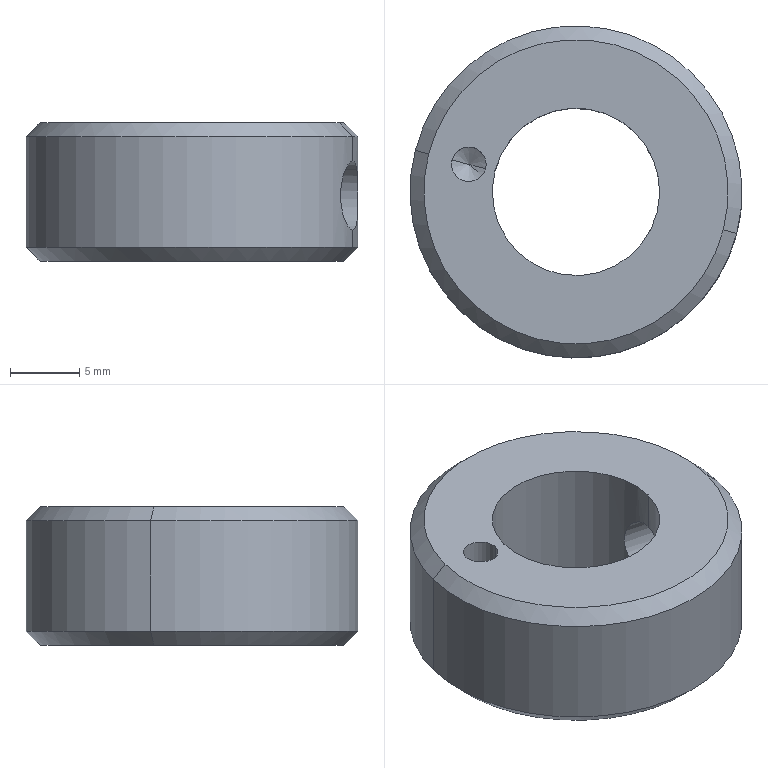Component | SolidWorks | TAR-02-036SpringFixingSleeve-1 | 1 solid | 16 faces | box 24 x 24 x 10 mm | volume 3147 mm3 | cylinder 8 | cone 6 | plane 2 | commonest cylinder face diameters 2.5 x2 5 x2 12.1 x2 24 x2
build123d program:
from build123d import *

# Parameters (mm, degrees)
SKETCH1_R                     = 12
SKETCH1_R_2                   = 6.05
BOSS_EXTRUDE1_DEPTH           = 10
CHAMFER1_SIZE                 = 1
M6_TAPPED_HOLE1_D             = 5
M6_TAPPED_HOLE1_DEPTH         = 12
M6_TAPPED_HOLE1_TIP           = 1.502
SIZE_MM_DOWEL_PIN_HOLE1_D     = 2.5
SIZE_MM_DOWEL_PIN_HOLE1_DEPTH = 7
SIZE_MM_DOWEL_PIN_HOLE1_TIP   = 0.7511


with BuildPart() as part:
    # Sketch1 → Boss-Extrude1 (new body)
    with BuildSketch(Plane.XY):
        Circle(SKETCH1_R)
        Circle(SKETCH1_R_2, mode=Mode.SUBTRACT)
    extrude(amount=BOSS_EXTRUDE1_DEPTH)

    # Chamfer1
    chamfer1_edges = [part.edges().sort_by_distance(p)[0] for p in [
        (-12, 0, 0),
        (-12, 0, 10),
    ]]
    chamfer(chamfer1_edges, length=CHAMFER1_SIZE)

    # M6 Tapped Hole1
    with Locations(Plane(origin=(12, 0, 4.747), x_dir=(0, 1, 0), z_dir=(1, 0, 0))):
        with Locations((0, 0)):
            Hole(M6_TAPPED_HOLE1_D / 2, depth=M6_TAPPED_HOLE1_DEPTH)
            with Locations((0, 0, -(M6_TAPPED_HOLE1_DEPTH + M6_TAPPED_HOLE1_TIP / 2))):  # 118° drill point
                Cone(0, M6_TAPPED_HOLE1_D / 2, M6_TAPPED_HOLE1_TIP, mode=Mode.SUBTRACT)

    # Size mm Dowel Pin Hole1
    with Locations(Plane(origin=(-8, 0, 10), x_dir=(1, 0, 0), z_dir=(0, 0, 1))):
        with Locations((0, 0)):
            Hole(SIZE_MM_DOWEL_PIN_HOLE1_D / 2, depth=SIZE_MM_DOWEL_PIN_HOLE1_DEPTH)
            with Locations((0, 0, -(SIZE_MM_DOWEL_PIN_HOLE1_DEPTH + SIZE_MM_DOWEL_PIN_HOLE1_TIP / 2))):  # 118° drill point
                Cone(0, SIZE_MM_DOWEL_PIN_HOLE1_D / 2, SIZE_MM_DOWEL_PIN_HOLE1_TIP, mode=Mode.SUBTRACT)


solid = part.part

# Placed as in the assembly
solid = solid.moved(Location((-45.891, 68.788, -66.881), (0, 0, -14.47)))
STEP:
#1=COLOUR_RGB('',0.7922,0.8196,0.9333);
#2=FILL_AREA_STYLE_COLOUR('',#1);
#3=FILL_AREA_STYLE('',(#2));
#4=SURFACE_STYLE_FILL_AREA(#3);
#5=SURFACE_SIDE_STYLE('',(#4));
#6=SURFACE_STYLE_USAGE(.BOTH.,#5);
#7=PRESENTATION_STYLE_ASSIGNMENT((#6));
#8=CARTESIAN_POINT('',(-2.159,2.799,-2.515));
#9=VERTEX_POINT('',#8);
#10=CARTESIAN_POINT('',(-2.064,2.775,-2.515));
#11=VERTEX_POINT('',#10);
#12=CARTESIAN_POINT('',(-2.112,2.787,-2.515));
#13=DIRECTION('',(0.,0.,1.));
#14=DIRECTION('',(0.9683,-0.2499,0.));
#15=AXIS2_PLACEMENT_3D('',#12,#13,#14);
#16=CIRCLE('',#15,0.04921);
#17=EDGE_CURVE('',#9,#11,#16,.T.);
#18=ORIENTED_EDGE('',*,*,#17,.F.);
#19=CARTESIAN_POINT('',(-2.159,2.799,-2.239));
#20=VERTEX_POINT('',#19);
#21=CARTESIAN_POINT('',(-2.159,2.799,-2.239));
#22=DIRECTION('',(0.,0.,1.));
#23=VECTOR('',#22,39.37);
#24=LINE('',#21,#23);
#25=EDGE_CURVE('',#9,#20,#24,.T.);
#26=ORIENTED_EDGE('',*,*,#25,.T.);
#27=CARTESIAN_POINT('',(-2.064,2.775,-2.239));
#28=VERTEX_POINT('',#27);
#29=CARTESIAN_POINT('',(-2.112,2.787,-2.239));
#30=DIRECTION('',(0.,0.,1.));
#31=DIRECTION('',(0.9683,-0.2499,0.));
#32=AXIS2_PLACEMENT_3D('',#29,#30,#31);
#33=CIRCLE('',#32,0.04921);
#34=EDGE_CURVE('',#20,#28,#33,.T.);
#35=ORIENTED_EDGE('',*,*,#34,.T.);
#36=CARTESIAN_POINT('',(-2.064,2.775,-2.239));
#37=DIRECTION('',(0.,0.,1.));
#38=VECTOR('',#37,39.37);
#39=LINE('',#36,#38);
#40=EDGE_CURVE('',#11,#28,#39,.T.);
#41=ORIENTED_EDGE('',*,*,#40,.F.);
#42=EDGE_LOOP('',(#18,#26,#35,#41));
#43=FACE_OUTER_BOUND('',#42,.T.);
#44=CARTESIAN_POINT('',(-2.112,2.787,-2.239));
#45=DIRECTION('',(0.,0.,1.));
#46=DIRECTION('',(0.9683,-0.2499,0.));
#47=AXIS2_PLACEMENT_3D('',#44,#45,#46);
#48=CYLINDRICAL_SURFACE('',#47,0.04921);
#49=ADVANCED_FACE('',(#43),#48,.F.);
#50=CARTESIAN_POINT('',(-2.112,2.787,-2.545));
#51=VERTEX_POINT('',#50);
#52=CARTESIAN_POINT('',(-2.064,2.775,-2.515));
#53=DIRECTION('',(0.83,-0.2142,0.515));
#54=VECTOR('',#53,39.37);
#55=LINE('',#52,#54);
#56=EDGE_CURVE('',#51,#11,#55,.T.);
#57=ORIENTED_EDGE('',*,*,#56,.F.);
#58=CARTESIAN_POINT('',(-2.159,2.799,-2.515));
#59=DIRECTION('',(-0.83,0.2142,0.515));
#60=VECTOR('',#59,39.37);
#61=LINE('',#58,#60);
#62=EDGE_CURVE('',#51,#9,#61,.T.);
#63=ORIENTED_EDGE('',*,*,#62,.T.);
#64=ORIENTED_EDGE('',*,*,#17,.T.);
#65=EDGE_LOOP('',(#57,#63,#64));
#66=FACE_OUTER_BOUND('',#65,.T.);
#67=CARTESIAN_POINT('',(-2.112,2.787,-2.515));
#68=DIRECTION('',(0.,0.,1.));
#69=DIRECTION('',(0.9683,-0.2499,0.));
#70=AXIS2_PLACEMENT_3D('',#67,#68,#69);
#71=CONICAL_SURFACE('',#70,0.04921,1.03);
#72=ADVANCED_FACE('',(#66),#71,.F.);
#73=CARTESIAN_POINT('',(-1.576,2.649,-2.545));
#74=VERTEX_POINT('',#73);
#75=CARTESIAN_POINT('',(-1.576,2.649,-2.348));
#76=VERTEX_POINT('',#75);
#77=CARTESIAN_POINT('',(-1.576,2.649,-2.545));
#78=CARTESIAN_POINT('',(-1.578,2.642,-2.545));
#79=CARTESIAN_POINT('',(-1.58,2.636,-2.544));
#80=CARTESIAN_POINT('',(-1.584,2.624,-2.541));
#81=CARTESIAN_POINT('',(-1.586,2.618,-2.54));
#82=CARTESIAN_POINT('',(-1.591,2.607,-2.535));
#83=CARTESIAN_POINT('',(-1.593,2.602,-2.532));
#84=CARTESIAN_POINT('',(-1.599,2.592,-2.524));
#85=CARTESIAN_POINT('',(-1.601,2.588,-2.52));
#86=CARTESIAN_POINT('',(-1.608,2.576,-2.507));
#87=CARTESIAN_POINT('',(-1.613,2.569,-2.496));
#88=CARTESIAN_POINT('',(-1.618,2.563,-2.478));
#89=CARTESIAN_POINT('',(-1.619,2.561,-2.472));
#90=CARTESIAN_POINT('',(-1.621,2.559,-2.459));
#91=CARTESIAN_POINT('',(-1.621,2.559,-2.453));
#92=CARTESIAN_POINT('',(-1.621,2.559,-2.44));
#93=CARTESIAN_POINT('',(-1.621,2.559,-2.433));
#94=CARTESIAN_POINT('',(-1.619,2.561,-2.42));
#95=CARTESIAN_POINT('',(-1.618,2.563,-2.414));
#96=CARTESIAN_POINT('',(-1.615,2.567,-2.402));
#97=CARTESIAN_POINT('',(-1.613,2.57,-2.397));
#98=CARTESIAN_POINT('',(-1.608,2.576,-2.386));
#99=CARTESIAN_POINT('',(-1.606,2.58,-2.381));
#100=CARTESIAN_POINT('',(-1.601,2.588,-2.372));
#101=CARTESIAN_POINT('',(-1.599,2.592,-2.368));
#102=CARTESIAN_POINT('',(-1.593,2.602,-2.361));
#103=CARTESIAN_POINT('',(-1.591,2.607,-2.358));
#104=CARTESIAN_POINT('',(-1.586,2.618,-2.353));
#105=CARTESIAN_POINT('',(-1.584,2.624,-2.351));
#106=CARTESIAN_POINT('',(-1.58,2.636,-2.348));
#107=CARTESIAN_POINT('',(-1.578,2.642,-2.348));
#108=CARTESIAN_POINT('',(-1.576,2.649,-2.348));
#109=B_SPLINE_CURVE_WITH_KNOTS('',3,(#77,#78,#79,#80,#81,#82,#83,#84,#85,#86,#87,#88,#89,#90,#91,#92,#93,#94,#95,#96,#97,#98,#99,#100,#101,#102,#103,#104,#105,#106,#107,#108),.UNSPECIFIED.,.F.,.F.,(4,2,2,2,2,2,2,2,2,2,2,2,2,2,2,4),(0.,0.0004941,0.0009882,0.001482,0.001976,0.002965,0.003459,0.003953,0.004447,0.004941,0.005435,0.005929,0.006423,0.006918,0.007412,0.007906),.UNSPECIFIED.);
#110=EDGE_CURVE('',#74,#76,#109,.T.);
#111=ORIENTED_EDGE('',*,*,#110,.T.);
#112=CARTESIAN_POINT('',(-1.349,2.59,-2.348));
#113=VERTEX_POINT('',#112);
#114=CARTESIAN_POINT('',(-1.349,2.59,-2.348));
#115=DIRECTION('',(0.9683,-0.2499,0.));
#116=VECTOR('',#115,39.37);
#117=LINE('',#114,#116);
#118=EDGE_CURVE('',#76,#113,#117,.T.);
#119=ORIENTED_EDGE('',*,*,#118,.T.);
#120=CARTESIAN_POINT('',(-1.349,2.59,-2.545));
#121=VERTEX_POINT('',#120);
#122=CARTESIAN_POINT('',(-1.349,2.59,-2.545));
#123=CARTESIAN_POINT('',(-1.351,2.584,-2.545));
#124=CARTESIAN_POINT('',(-1.353,2.578,-2.544));
#125=CARTESIAN_POINT('',(-1.356,2.566,-2.541));
#126=CARTESIAN_POINT('',(-1.358,2.56,-2.54));
#127=CARTESIAN_POINT('',(-1.362,2.548,-2.535));
#128=CARTESIAN_POINT('',(-1.364,2.543,-2.532));
#129=CARTESIAN_POINT('',(-1.368,2.533,-2.524));
#130=CARTESIAN_POINT('',(-1.37,2.528,-2.52));
#131=CARTESIAN_POINT('',(-1.375,2.516,-2.507));
#132=CARTESIAN_POINT('',(-1.378,2.509,-2.496));
#133=CARTESIAN_POINT('',(-1.382,2.502,-2.478));
#134=CARTESIAN_POINT('',(-1.382,2.5,-2.472));
#135=CARTESIAN_POINT('',(-1.384,2.498,-2.459));
#136=CARTESIAN_POINT('',(-1.384,2.497,-2.453));
#137=CARTESIAN_POINT('',(-1.384,2.497,-2.44));
#138=CARTESIAN_POINT('',(-1.384,2.498,-2.433));
#139=CARTESIAN_POINT('',(-1.382,2.5,-2.421));
#140=CARTESIAN_POINT('',(-1.382,2.502,-2.414));
#141=CARTESIAN_POINT('',(-1.379,2.507,-2.403));
#142=CARTESIAN_POINT('',(-1.378,2.509,-2.397));
#143=CARTESIAN_POINT('',(-1.375,2.516,-2.386));
#144=CARTESIAN_POINT('',(-1.373,2.52,-2.381));
#145=CARTESIAN_POINT('',(-1.37,2.528,-2.372));
#146=CARTESIAN_POINT('',(-1.368,2.533,-2.368));
#147=CARTESIAN_POINT('',(-1.364,2.543,-2.361));
#148=CARTESIAN_POINT('',(-1.362,2.548,-2.358));
#149=CARTESIAN_POINT('',(-1.358,2.56,-2.353));
#150=CARTESIAN_POINT('',(-1.356,2.565,-2.351));
#151=CARTESIAN_POINT('',(-1.353,2.578,-2.348));
#152=CARTESIAN_POINT('',(-1.351,2.584,-2.348));
#153=CARTESIAN_POINT('',(-1.349,2.59,-2.348));
#154=B_SPLINE_CURVE_WITH_KNOTS('',3,(#122,#123,#124,#125,#126,#127,#128,#129,#130,#131,#132,#133,#134,#135,#136,#137,#138,#139,#140,#141,#142,#143,#144,#145,#146,#147,#148,#149,#150,#151,#152,#153),.UNSPECIFIED.,.F.,.F.,(4,2,2,2,2,2,2,2,2,2,2,2,2,2,2,4),(0.,0.0004899,0.0009797,0.00147,0.001959,0.002939,0.003429,0.003919,0.004409,0.004899,0.005388,0.005878,0.006368,0.006858,0.007348,0.007838),.UNSPECIFIED.);
#155=EDGE_CURVE('',#121,#113,#154,.T.);
#156=ORIENTED_EDGE('',*,*,#155,.F.);
#157=CARTESIAN_POINT('',(-1.349,2.59,-2.545));
#158=DIRECTION('',(0.9683,-0.2499,0.));
#159=VECTOR('',#158,39.37);
#160=LINE('',#157,#159);
#161=EDGE_CURVE('',#74,#121,#160,.T.);
#162=ORIENTED_EDGE('',*,*,#161,.F.);
#163=EDGE_LOOP('',(#111,#119,#156,#162));
#164=FACE_OUTER_BOUND('',#163,.T.);
#165=CARTESIAN_POINT('',(-1.349,2.59,-2.446));
#166=DIRECTION('',(0.9683,-0.2499,0.));
#167=DIRECTION('',(0.,0.,-1.));
#168=AXIS2_PLACEMENT_3D('',#165,#166,#167);
#169=CYLINDRICAL_SURFACE('',#168,0.09843);
#170=ADVANCED_FACE('',(#164),#169,.F.);
#171=CARTESIAN_POINT('',(-1.387,2.6,-2.239));
#172=VERTEX_POINT('',#171);
#173=CARTESIAN_POINT('',(-2.226,2.816,-2.239));
#174=VERTEX_POINT('',#173);
#175=CARTESIAN_POINT('',(-1.807,2.708,-2.239));
#176=DIRECTION('',(0.,0.,1.));
#177=DIRECTION('',(0.9683,-0.2499,0.));
#178=AXIS2_PLACEMENT_3D('',#175,#176,#177);
#179=CIRCLE('',#178,0.4331);
#180=EDGE_CURVE('',#172,#174,#179,.T.);
#181=ORIENTED_EDGE('',*,*,#180,.F.);
#182=CARTESIAN_POINT('',(-1.349,2.59,-2.279));
#183=VERTEX_POINT('',#182);
#184=CARTESIAN_POINT('',(-1.387,2.6,-2.239));
#185=DIRECTION('',(0.6847,-0.1767,-0.7071));
#186=VECTOR('',#185,39.37);
#187=LINE('',#184,#186);
#188=EDGE_CURVE('',#172,#183,#187,.T.);
#189=ORIENTED_EDGE('',*,*,#188,.T.);
#190=CARTESIAN_POINT('',(-2.264,2.826,-2.279));
#191=VERTEX_POINT('',#190);
#192=CARTESIAN_POINT('',(-1.807,2.708,-2.279));
#193=DIRECTION('',(0.,0.,-1.));
#194=DIRECTION('',(0.9683,-0.2499,0.));
#195=AXIS2_PLACEMENT_3D('',#192,#193,#194);
#196=CIRCLE('',#195,0.4724);
#197=EDGE_CURVE('',#191,#183,#196,.T.);
#198=ORIENTED_EDGE('',*,*,#197,.F.);
#199=CARTESIAN_POINT('',(-2.226,2.816,-2.239));
#200=DIRECTION('',(-0.6847,0.1767,-0.7071));
#201=VECTOR('',#200,39.37);
#202=LINE('',#199,#201);
#203=EDGE_CURVE('',#174,#191,#202,.T.);
#204=ORIENTED_EDGE('',*,*,#203,.F.);
#205=EDGE_LOOP('',(#181,#189,#198,#204));
#206=FACE_OUTER_BOUND('',#205,.T.);
#207=CARTESIAN_POINT('',(-1.807,2.708,-2.239));
#208=DIRECTION('',(0.,0.,-1.));
#209=DIRECTION('',(-0.9683,0.2499,0.));
#210=AXIS2_PLACEMENT_3D('',#207,#208,#209);
#211=CONICAL_SURFACE('',#210,0.4331,0.7854);
#212=ADVANCED_FACE('',(#206),#211,.T.);
#213=CARTESIAN_POINT('',(-2.226,2.816,-2.633));
#214=VERTEX_POINT('',#213);
#215=CARTESIAN_POINT('',(-1.387,2.6,-2.633));
#216=VERTEX_POINT('',#215);
#217=CARTESIAN_POINT('',(-1.807,2.708,-2.633));
#218=DIRECTION('',(0.,0.,-1.));
#219=DIRECTION('',(0.9683,-0.2499,0.));
#220=AXIS2_PLACEMENT_3D('',#217,#218,#219);
#221=CIRCLE('',#220,0.4331);
#222=EDGE_CURVE('',#214,#216,#221,.T.);
#223=ORIENTED_EDGE('',*,*,#222,.F.);
#224=CARTESIAN_POINT('',(-2.264,2.826,-2.594));
#225=VERTEX_POINT('',#224);
#226=CARTESIAN_POINT('',(-2.264,2.826,-2.594));
#227=DIRECTION('',(-0.6847,0.1767,0.7071));
#228=VECTOR('',#227,39.37);
#229=LINE('',#226,#228);
#230=EDGE_CURVE('',#214,#225,#229,.T.);
#231=ORIENTED_EDGE('',*,*,#230,.T.);
#232=CARTESIAN_POINT('',(-1.349,2.59,-2.594));
#233=VERTEX_POINT('',#232);
#234=CARTESIAN_POINT('',(-1.807,2.708,-2.594));
#235=DIRECTION('',(0.,0.,1.));
#236=DIRECTION('',(0.9683,-0.2499,0.));
#237=AXIS2_PLACEMENT_3D('',#234,#235,#236);
#238=CIRCLE('',#237,0.4724);
#239=EDGE_CURVE('',#233,#225,#238,.T.);
#240=ORIENTED_EDGE('',*,*,#239,.F.);
#241=CARTESIAN_POINT('',(-1.349,2.59,-2.594));
#242=DIRECTION('',(0.6847,-0.1767,0.7071));
#243=VECTOR('',#242,39.37);
#244=LINE('',#241,#243);
#245=EDGE_CURVE('',#216,#233,#244,.T.);
#246=ORIENTED_EDGE('',*,*,#245,.F.);
#247=EDGE_LOOP('',(#223,#231,#240,#246));
#248=FACE_OUTER_BOUND('',#247,.T.);
#249=CARTESIAN_POINT('',(-1.807,2.708,-2.594));
#250=DIRECTION('',(0.,0.,1.));
#251=DIRECTION('',(0.9683,-0.2499,0.));
#252=AXIS2_PLACEMENT_3D('',#249,#250,#251);
#253=CONICAL_SURFACE('',#252,0.4724,0.7854);
#254=ADVANCED_FACE('',(#248),#253,.T.);
#255=CARTESIAN_POINT('',(-2.037,2.768,-2.239));
#256=VERTEX_POINT('',#255);
#257=CARTESIAN_POINT('',(-1.576,2.649,-2.239));
#258=VERTEX_POINT('',#257);
#259=CARTESIAN_POINT('',(-1.807,2.708,-2.239));
#260=DIRECTION('',(0.,0.,1.));
#261=DIRECTION('',(0.9683,-0.2499,0.));
#262=AXIS2_PLACEMENT_3D('',#259,#260,#261);
#263=CIRCLE('',#262,0.2382);
#264=EDGE_CURVE('',#256,#258,#263,.T.);
#265=ORIENTED_EDGE('',*,*,#264,.T.);
#266=CARTESIAN_POINT('',(-1.576,2.649,-2.239));
#267=DIRECTION('',(0.,0.,-1.));
#268=VECTOR('',#267,39.37);
#269=LINE('',#266,#268);
#270=EDGE_CURVE('',#258,#76,#269,.T.);
#271=ORIENTED_EDGE('',*,*,#270,.T.);
#272=ORIENTED_EDGE('',*,*,#110,.F.);
#273=CARTESIAN_POINT('',(-1.576,2.649,-2.633));
#274=VERTEX_POINT('',#273);
#275=CARTESIAN_POINT('',(-1.576,2.649,-2.239));
#276=DIRECTION('',(0.,0.,-1.));
#277=VECTOR('',#276,39.37);
#278=LINE('',#275,#277);
#279=EDGE_CURVE('',#74,#274,#278,.T.);
#280=ORIENTED_EDGE('',*,*,#279,.T.);
#281=CARTESIAN_POINT('',(-2.037,2.768,-2.633));
#282=VERTEX_POINT('',#281);
#283=CARTESIAN_POINT('',(-1.807,2.708,-2.633));
#284=DIRECTION('',(0.,0.,1.));
#285=DIRECTION('',(0.9683,-0.2499,0.));
#286=AXIS2_PLACEMENT_3D('',#283,#284,#285);
#287=CIRCLE('',#286,0.2382);
#288=EDGE_CURVE('',#282,#274,#287,.T.);
#289=ORIENTED_EDGE('',*,*,#288,.F.);
#290=CARTESIAN_POINT('',(-2.037,2.768,-2.239));
#291=DIRECTION('',(0.,0.,-1.));
#292=VECTOR('',#291,39.37);
#293=LINE('',#290,#292);
#294=EDGE_CURVE('',#256,#282,#293,.T.);
#295=ORIENTED_EDGE('',*,*,#294,.F.);
#296=EDGE_LOOP('',(#265,#271,#272,#280,#289,#295));
#297=FACE_OUTER_BOUND('',#296,.T.);
#298=CARTESIAN_POINT('',(-1.807,2.708,-2.239));
#299=DIRECTION('',(0.,0.,-1.));
#300=DIRECTION('',(-0.9683,0.2499,0.));
#301=AXIS2_PLACEMENT_3D('',#298,#299,#300);
#302=CYLINDRICAL_SURFACE('',#301,0.2382);
#303=ADVANCED_FACE('',(#297),#302,.F.);
#304=ORIENTED_EDGE('',*,*,#197,.T.);
#305=CARTESIAN_POINT('',(-1.349,2.59,-2.239));
#306=DIRECTION('',(0.,0.,-1.));
#307=VECTOR('',#306,39.37);
#308=LINE('',#305,#307);
#309=EDGE_CURVE('',#183,#113,#308,.T.);
#310=ORIENTED_EDGE('',*,*,#309,.T.);
#311=CARTESIAN_POINT('',(-1.349,2.59,-2.348));
#312=CARTESIAN_POINT('',(-1.346,2.603,-2.348));
#313=CARTESIAN_POINT('',(-1.343,2.615,-2.35));
#314=CARTESIAN_POINT('',(-1.34,2.633,-2.358));
#315=CARTESIAN_POINT('',(-1.339,2.639,-2.361));
#316=CARTESIAN_POINT('',(-1.338,2.649,-2.368));
#317=CARTESIAN_POINT('',(-1.337,2.654,-2.372));
#318=CARTESIAN_POINT('',(-1.336,2.663,-2.381));
#319=CARTESIAN_POINT('',(-1.336,2.668,-2.386));
#320=CARTESIAN_POINT('',(-1.335,2.675,-2.397));
#321=CARTESIAN_POINT('',(-1.335,2.678,-2.402));
#322=CARTESIAN_POINT('',(-1.335,2.685,-2.42));
#323=CARTESIAN_POINT('',(-1.335,2.688,-2.433));
#324=CARTESIAN_POINT('',(-1.335,2.688,-2.453));
#325=CARTESIAN_POINT('',(-1.335,2.687,-2.459));
#326=CARTESIAN_POINT('',(-1.335,2.685,-2.472));
#327=CARTESIAN_POINT('',(-1.335,2.683,-2.478));
#328=CARTESIAN_POINT('',(-1.335,2.678,-2.49));
#329=CARTESIAN_POINT('',(-1.335,2.675,-2.496));
#330=CARTESIAN_POINT('',(-1.336,2.668,-2.506));
#331=CARTESIAN_POINT('',(-1.336,2.663,-2.511));
#332=CARTESIAN_POINT('',(-1.338,2.65,-2.525));
#333=CARTESIAN_POINT('',(-1.339,2.639,-2.532));
#334=CARTESIAN_POINT('',(-1.342,2.621,-2.54));
#335=CARTESIAN_POINT('',(-1.343,2.615,-2.541));
#336=CARTESIAN_POINT('',(-1.346,2.603,-2.544));
#337=CARTESIAN_POINT('',(-1.348,2.596,-2.545));
#338=CARTESIAN_POINT('',(-1.349,2.59,-2.545));
#339=B_SPLINE_CURVE_WITH_KNOTS('',3,(#311,#312,#313,#314,#315,#316,#317,#318,#319,#320,#321,#322,#323,#324,#325,#326,#327,#328,#329,#330,#331,#332,#333,#334,#335,#336,#337,#338),.UNSPECIFIED.,.F.,.F.,(4,2,2,2,2,2,2,2,2,2,2,2,2,4),(0.007838,0.008817,0.009307,0.009797,0.01029,0.01078,0.01176,0.01225,0.01273,0.01322,0.01371,0.01469,0.01518,0.01567),.UNSPECIFIED.);
#340=EDGE_CURVE('',#113,#121,#339,.T.);
#341=ORIENTED_EDGE('',*,*,#340,.T.);
#342=CARTESIAN_POINT('',(-1.349,2.59,-2.239));
#343=DIRECTION('',(0.,0.,-1.));
#344=VECTOR('',#343,39.37);
#345=LINE('',#342,#344);
#346=EDGE_CURVE('',#121,#233,#345,.T.);
#347=ORIENTED_EDGE('',*,*,#346,.T.);
#348=ORIENTED_EDGE('',*,*,#239,.T.);
#349=CARTESIAN_POINT('',(-2.264,2.826,-2.239));
#350=DIRECTION('',(0.,0.,-1.));
#351=VECTOR('',#350,39.37);
#352=LINE('',#349,#351);
#353=EDGE_CURVE('',#191,#225,#352,.T.);
#354=ORIENTED_EDGE('',*,*,#353,.F.);
#355=EDGE_LOOP('',(#304,#310,#341,#347,#348,#354));
#356=FACE_OUTER_BOUND('',#355,.T.);
#357=CARTESIAN_POINT('',(-1.807,2.708,-2.239));
#358=DIRECTION('',(0.,0.,-1.));
#359=DIRECTION('',(-0.9683,0.2499,0.));
#360=AXIS2_PLACEMENT_3D('',#357,#358,#359);
#361=CYLINDRICAL_SURFACE('',#360,0.4724);
#362=ADVANCED_FACE('',(#356),#361,.T.);
#363=CARTESIAN_POINT('',(-2.112,2.787,-2.239));
#364=DIRECTION('',(0.,0.,1.));
#365=DIRECTION('',(0.9683,-0.2499,0.));
#366=AXIS2_PLACEMENT_3D('',#363,#364,#365);
#367=CIRCLE('',#366,0.04921);
#368=EDGE_CURVE('',#28,#20,#367,.T.);
#369=ORIENTED_EDGE('',*,*,#368,.F.);
#370=ORIENTED_EDGE('',*,*,#34,.F.);
#371=EDGE_LOOP('',(#369,#370));
#372=FACE_BOUND('',#371,.T.);
#373=CARTESIAN_POINT('',(-1.807,2.708,-2.239));
#374=DIRECTION('',(0.,0.,1.));
#375=DIRECTION('',(0.9683,-0.2499,0.));
#376=AXIS2_PLACEMENT_3D('',#373,#374,#375);
#377=CIRCLE('',#376,0.4331);
#378=EDGE_CURVE('',#174,#172,#377,.T.);
#379=ORIENTED_EDGE('',*,*,#378,.T.);
#380=ORIENTED_EDGE('',*,*,#180,.T.);
#381=EDGE_LOOP('',(#379,#380));
#382=FACE_OUTER_BOUND('',#381,.T.);
#383=ORIENTED_EDGE('',*,*,#264,.F.);
#384=CARTESIAN_POINT('',(-1.807,2.708,-2.239));
#385=DIRECTION('',(0.,0.,1.));
#386=DIRECTION('',(0.9683,-0.2499,0.));
#387=AXIS2_PLACEMENT_3D('',#384,#385,#386);
#388=CIRCLE('',#387,0.2382);
#389=EDGE_CURVE('',#258,#256,#388,.T.);
#390=ORIENTED_EDGE('',*,*,#389,.F.);
#391=EDGE_LOOP('',(#383,#390));
#392=FACE_BOUND('',#391,.T.);
#393=CARTESIAN_POINT('',(-1.807,2.708,-2.239));
#394=DIRECTION('',(0.,0.,1.));
#395=DIRECTION('',(0.9683,-0.2499,0.));
#396=AXIS2_PLACEMENT_3D('',#393,#394,#395);
#397=PLANE('',#396);
#398=ADVANCED_FACE('',(#372,#382,#392),#397,.T.);
#399=CARTESIAN_POINT('',(-1.807,2.708,-2.633));
#400=DIRECTION('',(0.,0.,-1.));
#401=DIRECTION('',(0.9683,-0.2499,0.));
#402=AXIS2_PLACEMENT_3D('',#399,#400,#401);
#403=CIRCLE('',#402,0.4331);
#404=EDGE_CURVE('',#216,#214,#403,.T.);
#405=ORIENTED_EDGE('',*,*,#404,.T.);
#406=ORIENTED_EDGE('',*,*,#222,.T.);
#407=EDGE_LOOP('',(#405,#406));
#408=FACE_OUTER_BOUND('',#407,.T.);
#409=ORIENTED_EDGE('',*,*,#288,.T.);
#410=CARTESIAN_POINT('',(-1.807,2.708,-2.633));
#411=DIRECTION('',(0.,0.,1.));
#412=DIRECTION('',(0.9683,-0.2499,0.));
#413=AXIS2_PLACEMENT_3D('',#410,#411,#412);
#414=CIRCLE('',#413,0.2382);
#415=EDGE_CURVE('',#274,#282,#414,.T.);
#416=ORIENTED_EDGE('',*,*,#415,.T.);
#417=EDGE_LOOP('',(#409,#416));
#418=FACE_BOUND('',#417,.T.);
#419=CARTESIAN_POINT('',(-1.807,2.708,-2.633));
#420=DIRECTION('',(0.,0.,1.));
#421=DIRECTION('',(0.9683,-0.2499,0.));
#422=AXIS2_PLACEMENT_3D('',#419,#420,#421);
#423=PLANE('',#422);
#424=ADVANCED_FACE('',(#408,#418),#423,.F.);
#425=ORIENTED_EDGE('',*,*,#309,.F.);
#426=CARTESIAN_POINT('',(-1.807,2.708,-2.279));
#427=DIRECTION('',(0.,0.,-1.));
#428=DIRECTION('',(0.9683,-0.2499,0.));
#429=AXIS2_PLACEMENT_3D('',#426,#427,#428);
#430=CIRCLE('',#429,0.4724);
#431=EDGE_CURVE('',#183,#191,#430,.T.);
#432=ORIENTED_EDGE('',*,*,#431,.T.);
#433=ORIENTED_EDGE('',*,*,#353,.T.);
#434=CARTESIAN_POINT('',(-1.807,2.708,-2.594));
#435=DIRECTION('',(0.,0.,1.));
#436=DIRECTION('',(0.9683,-0.2499,0.));
#437=AXIS2_PLACEMENT_3D('',#434,#435,#436);
#438=CIRCLE('',#437,0.4724);
#439=EDGE_CURVE('',#225,#233,#438,.T.);
#440=ORIENTED_EDGE('',*,*,#439,.T.);
#441=ORIENTED_EDGE('',*,*,#346,.F.);
#442=ORIENTED_EDGE('',*,*,#155,.T.);
#443=EDGE_LOOP('',(#425,#432,#433,#440,#441,#442));
#444=FACE_OUTER_BOUND('',#443,.T.);
#445=CARTESIAN_POINT('',(-1.807,2.708,-2.239));
#446=DIRECTION('',(0.,0.,-1.));
#447=DIRECTION('',(-0.9683,0.2499,0.));
#448=AXIS2_PLACEMENT_3D('',#445,#446,#447);
#449=CYLINDRICAL_SURFACE('',#448,0.4724);
#450=ADVANCED_FACE('',(#444),#449,.T.);
#451=ORIENTED_EDGE('',*,*,#270,.F.);
#452=ORIENTED_EDGE('',*,*,#389,.T.);
#453=ORIENTED_EDGE('',*,*,#294,.T.);
#454=ORIENTED_EDGE('',*,*,#415,.F.);
#455=ORIENTED_EDGE('',*,*,#279,.F.);
#456=CARTESIAN_POINT('',(-1.576,2.649,-2.348));
#457=CARTESIAN_POINT('',(-1.574,2.655,-2.348));
#458=CARTESIAN_POINT('',(-1.573,2.661,-2.348));
#459=CARTESIAN_POINT('',(-1.571,2.674,-2.351));
#460=CARTESIAN_POINT('',(-1.57,2.68,-2.353));
#461=CARTESIAN_POINT('',(-1.569,2.692,-2.358));
#462=CARTESIAN_POINT('',(-1.569,2.698,-2.361));
#463=CARTESIAN_POINT('',(-1.568,2.709,-2.368));
#464=CARTESIAN_POINT('',(-1.569,2.714,-2.372));
#465=CARTESIAN_POINT('',(-1.569,2.723,-2.381));
#466=CARTESIAN_POINT('',(-1.569,2.728,-2.386));
#467=CARTESIAN_POINT('',(-1.57,2.735,-2.397));
#468=CARTESIAN_POINT('',(-1.57,2.738,-2.402));
#469=CARTESIAN_POINT('',(-1.571,2.744,-2.414));
#470=CARTESIAN_POINT('',(-1.572,2.746,-2.42));
#471=CARTESIAN_POINT('',(-1.572,2.749,-2.433));
#472=CARTESIAN_POINT('',(-1.572,2.749,-2.44));
#473=CARTESIAN_POINT('',(-1.572,2.749,-2.459));
#474=CARTESIAN_POINT('',(-1.572,2.746,-2.472));
#475=CARTESIAN_POINT('',(-1.57,2.738,-2.49));
#476=CARTESIAN_POINT('',(-1.57,2.735,-2.496));
#477=CARTESIAN_POINT('',(-1.569,2.728,-2.506));
#478=CARTESIAN_POINT('',(-1.569,2.723,-2.511));
#479=CARTESIAN_POINT('',(-1.569,2.714,-2.52));
#480=CARTESIAN_POINT('',(-1.568,2.709,-2.524));
#481=CARTESIAN_POINT('',(-1.569,2.698,-2.531));
#482=CARTESIAN_POINT('',(-1.569,2.692,-2.535));
#483=CARTESIAN_POINT('',(-1.57,2.68,-2.54));
#484=CARTESIAN_POINT('',(-1.571,2.674,-2.541));
#485=CARTESIAN_POINT('',(-1.573,2.661,-2.544));
#486=CARTESIAN_POINT('',(-1.574,2.655,-2.545));
#487=CARTESIAN_POINT('',(-1.576,2.649,-2.545));
#488=B_SPLINE_CURVE_WITH_KNOTS('',3,(#456,#457,#458,#459,#460,#461,#462,#463,#464,#465,#466,#467,#468,#469,#470,#471,#472,#473,#474,#475,#476,#477,#478,#479,#480,#481,#482,#483,#484,#485,#486,#487),.UNSPECIFIED.,.F.,.F.,(4,2,2,2,2,2,2,2,2,2,2,2,2,2,2,4),(0.007906,0.0084,0.008893,0.009387,0.009881,0.01037,0.01087,0.01136,0.01186,0.01284,0.01334,0.01383,0.01432,0.01482,0.01531,0.01581),.UNSPECIFIED.);
#489=EDGE_CURVE('',#76,#74,#488,.T.);
#490=ORIENTED_EDGE('',*,*,#489,.F.);
#491=EDGE_LOOP('',(#451,#452,#453,#454,#455,#490));
#492=FACE_OUTER_BOUND('',#491,.T.);
#493=CARTESIAN_POINT('',(-1.807,2.708,-2.239));
#494=DIRECTION('',(0.,0.,-1.));
#495=DIRECTION('',(-0.9683,0.2499,0.));
#496=AXIS2_PLACEMENT_3D('',#493,#494,#495);
#497=CYLINDRICAL_SURFACE('',#496,0.2382);
#498=ADVANCED_FACE('',(#492),#497,.F.);
#499=ORIENTED_EDGE('',*,*,#230,.F.);
#500=ORIENTED_EDGE('',*,*,#404,.F.);
#501=ORIENTED_EDGE('',*,*,#245,.T.);
#502=ORIENTED_EDGE('',*,*,#439,.F.);
#503=EDGE_LOOP('',(#499,#500,#501,#502));
#504=FACE_OUTER_BOUND('',#503,.T.);
#505=CARTESIAN_POINT('',(-1.807,2.708,-2.594));
#506=DIRECTION('',(0.,0.,1.));
#507=DIRECTION('',(0.9683,-0.2499,0.));
#508=AXIS2_PLACEMENT_3D('',#505,#506,#507);
#509=CONICAL_SURFACE('',#508,0.4724,0.7854);
#510=ADVANCED_FACE('',(#504),#509,.T.);
#511=ORIENTED_EDGE('',*,*,#188,.F.);
#512=ORIENTED_EDGE('',*,*,#378,.F.);
#513=ORIENTED_EDGE('',*,*,#203,.T.);
#514=ORIENTED_EDGE('',*,*,#431,.F.);
#515=EDGE_LOOP('',(#511,#512,#513,#514));
#516=FACE_OUTER_BOUND('',#515,.T.);
#517=CARTESIAN_POINT('',(-1.807,2.708,-2.239));
#518=DIRECTION('',(0.,0.,-1.));
#519=DIRECTION('',(-0.9683,0.2499,0.));
#520=AXIS2_PLACEMENT_3D('',#517,#518,#519);
#521=CONICAL_SURFACE('',#520,0.4331,0.7854);
#522=ADVANCED_FACE('',(#516),#521,.T.);
#523=ORIENTED_EDGE('',*,*,#118,.F.);
#524=ORIENTED_EDGE('',*,*,#489,.T.);
#525=ORIENTED_EDGE('',*,*,#161,.T.);
#526=ORIENTED_EDGE('',*,*,#340,.F.);
#527=EDGE_LOOP('',(#523,#524,#525,#526));
#528=FACE_OUTER_BOUND('',#527,.T.);
#529=CARTESIAN_POINT('',(-1.349,2.59,-2.446));
#530=DIRECTION('',(0.9683,-0.2499,0.));
#531=DIRECTION('',(0.,0.,-1.));
#532=AXIS2_PLACEMENT_3D('',#529,#530,#531);
#533=CYLINDRICAL_SURFACE('',#532,0.09843);
#534=ADVANCED_FACE('',(#528),#533,.F.);
#535=ORIENTED_EDGE('',*,*,#62,.F.);
#536=ORIENTED_EDGE('',*,*,#56,.T.);
#537=CARTESIAN_POINT('',(-2.112,2.787,-2.515));
#538=DIRECTION('',(0.,0.,1.));
#539=DIRECTION('',(0.9683,-0.2499,0.));
#540=AXIS2_PLACEMENT_3D('',#537,#538,#539);
#541=CIRCLE('',#540,0.04921);
#542=EDGE_CURVE('',#11,#9,#541,.T.);
#543=ORIENTED_EDGE('',*,*,#542,.T.);
#544=EDGE_LOOP('',(#535,#536,#543));
#545=FACE_OUTER_BOUND('',#544,.T.);
#546=CARTESIAN_POINT('',(-2.112,2.787,-2.515));
#547=DIRECTION('',(0.,0.,1.));
#548=DIRECTION('',(0.9683,-0.2499,0.));
#549=AXIS2_PLACEMENT_3D('',#546,#547,#548);
#550=CONICAL_SURFACE('',#549,0.04921,1.03);
#551=ADVANCED_FACE('',(#545),#550,.F.);
#552=ORIENTED_EDGE('',*,*,#25,.F.);
#553=ORIENTED_EDGE('',*,*,#542,.F.);
#554=ORIENTED_EDGE('',*,*,#40,.T.);
#555=ORIENTED_EDGE('',*,*,#368,.T.);
#556=EDGE_LOOP('',(#552,#553,#554,#555));
#557=FACE_OUTER_BOUND('',#556,.T.);
#558=CARTESIAN_POINT('',(-2.112,2.787,-2.239));
#559=DIRECTION('',(0.,0.,1.));
#560=DIRECTION('',(0.9683,-0.2499,0.));
#561=AXIS2_PLACEMENT_3D('',#558,#559,#560);
#562=CYLINDRICAL_SURFACE('',#561,0.04921);
#563=ADVANCED_FACE('',(#557),#562,.F.);
#564=CLOSED_SHELL('',(#49,#72,#170,#212,#254,#303,#362,#398,#424,#450,#498,#510,#522,#534,#551,#563));
#565=MANIFOLD_SOLID_BREP('',#564);
#566=STYLED_ITEM('',(#7),#565);
#567=PRESENTATION_LAYER_ASSIGNMENT('','',(#566));
#568=CARTESIAN_POINT('',(0.,0.,0.));
#569=DIRECTION('',(0.,0.,1.));
#570=DIRECTION('',(1.,0.,0.));
#571=AXIS2_PLACEMENT_3D('',#568,#569,#570);
#572=(LENGTH_UNIT()NAMED_UNIT(*)SI_UNIT($,.METRE.));
#573=LENGTH_MEASURE_WITH_UNIT(LENGTH_MEASURE(0.0254),#572);
#574=DIMENSIONAL_EXPONENTS(1.,0.,0.,0.,0.,0.,0.);
#575=(CONVERSION_BASED_UNIT('',#573)LENGTH_UNIT()NAMED_UNIT(#574));
#576=UNCERTAINTY_MEASURE_WITH_UNIT(LENGTH_MEASURE(0.00001),#575,'','');
#577=(NAMED_UNIT(*)PLANE_ANGLE_UNIT()SI_UNIT($,.RADIAN.));
#578=(NAMED_UNIT(*)SI_UNIT($,.STERADIAN.)SOLID_ANGLE_UNIT());
#579=(GEOMETRIC_REPRESENTATION_CONTEXT(3)GLOBAL_UNCERTAINTY_ASSIGNED_CONTEXT((#576))GLOBAL_UNIT_ASSIGNED_CONTEXT((#575,#577,#578))REPRESENTATION_CONTEXT('',''));
#580=ADVANCED_BREP_SHAPE_REPRESENTATION('',(#565,#571),#579);
#581=(LENGTH_UNIT()NAMED_UNIT(*)SI_UNIT($,.METRE.));
#582=LENGTH_MEASURE_WITH_UNIT(LENGTH_MEASURE(0.0254),#581);
#583=DIMENSIONAL_EXPONENTS(1.,0.,0.,0.,0.,0.,0.);
#584=(CONVERSION_BASED_UNIT('',#582)LENGTH_UNIT()NAMED_UNIT(#583));
#585=UNCERTAINTY_MEASURE_WITH_UNIT(LENGTH_MEASURE(0.00001),#584,'','');
#586=(NAMED_UNIT(*)PLANE_ANGLE_UNIT()SI_UNIT($,.RADIAN.));
#587=(NAMED_UNIT(*)SI_UNIT($,.STERADIAN.)SOLID_ANGLE_UNIT());
#588=(GEOMETRIC_REPRESENTATION_CONTEXT(3)GLOBAL_UNCERTAINTY_ASSIGNED_CONTEXT((#585))GLOBAL_UNIT_ASSIGNED_CONTEXT((#584,#586,#587))REPRESENTATION_CONTEXT('',''));
#589=MECHANICAL_DESIGN_GEOMETRIC_PRESENTATION_REPRESENTATION('',(#566),#588);